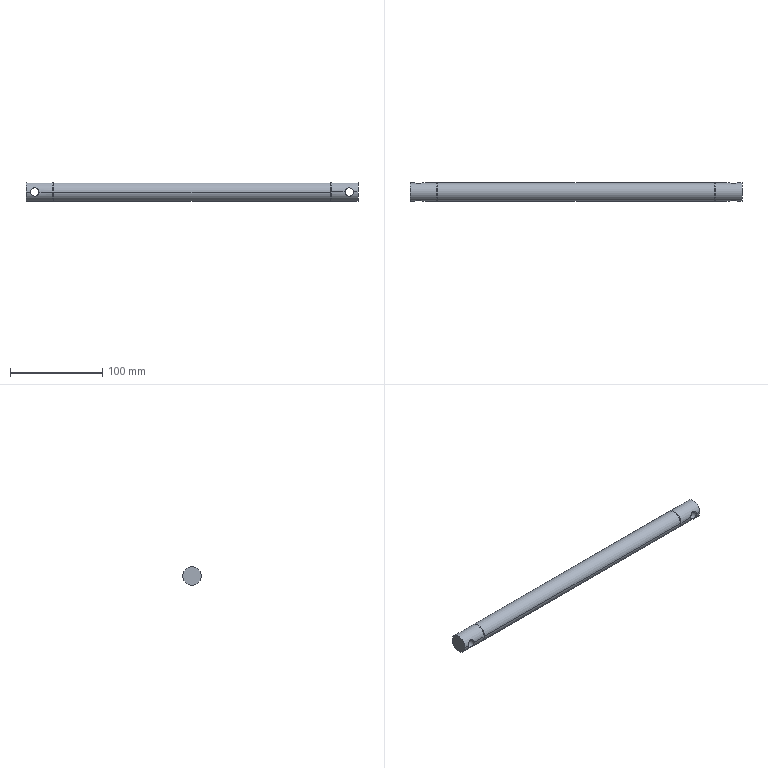Component | SolidWorks | DrivenShaft-1 | 1 solid | 20 faces | box 360 x 20 x 20 mm | volume 110558 mm3 | cylinder 14 | plane 6 | commonest cylinder face diameters 20 x6 9 x4 19 x4
build123d program:
from build123d import *

# Parameters (mm, degrees)
F_9_0_9_DIAMETER_HOLE1_D = 9


with BuildPart() as part:
    # Sketch1 → Revolve1 (revolve)
    with BuildSketch(Plane.XY, mode=Mode.PRIVATE) as revolve1_sk:
        Polygon((0, 0), (360, 0), (360, 10), (331, 10), (331, 9.5), (330, 9.5), (330, 10), (30, 10), (30, 9.5), (29, 9.5), (29, 10), (0, 10), align=None)
    revolve(revolve1_sk.sketch.rotate(Axis((0, 0, 0), (1, 0, 0)), 90), axis=Axis((0, 0, 0), (1, 0, 0)))

    # 9.0 _9_ Diameter Hole1 (through all)
    with Locations(Plane.XY.offset(10)):
        with Locations((9.5, 0), (350.5, 0)):
            Hole(F_9_0_9_DIAMETER_HOLE1_D / 2)


solid = part.part

# Placed as in the assembly
solid = solid.moved(Location((5755.006, 3057.679, 47.375), (90, 0, 0)))
STEP:
#1=COLOUR_RGB('',0.7922,0.8196,0.9333);
#2=FILL_AREA_STYLE_COLOUR('',#1);
#3=FILL_AREA_STYLE('',(#2));
#4=SURFACE_STYLE_FILL_AREA(#3);
#5=SURFACE_SIDE_STYLE('',(#4));
#6=SURFACE_STYLE_USAGE(.BOTH.,#5);
#7=PRESENTATION_STYLE_ASSIGNMENT((#6));
#8=CARTESIAN_POINT('',(240.551,119.987,1.865));
#9=VERTEX_POINT('',#8);
#10=CARTESIAN_POINT('',(240.197,119.987,1.865));
#11=VERTEX_POINT('',#10);
#12=CARTESIAN_POINT('',(240.551,119.987,1.865));
#13=CARTESIAN_POINT('',(240.551,119.987,1.853));
#14=CARTESIAN_POINT('',(240.55,119.988,1.842));
#15=CARTESIAN_POINT('',(240.546,119.99,1.819));
#16=CARTESIAN_POINT('',(240.542,119.991,1.808));
#17=CARTESIAN_POINT('',(240.533,119.995,1.786));
#18=CARTESIAN_POINT('',(240.528,119.998,1.776));
#19=CARTESIAN_POINT('',(240.515,120.002,1.757));
#20=CARTESIAN_POINT('',(240.508,120.005,1.748));
#21=CARTESIAN_POINT('',(240.491,120.011,1.732));
#22=CARTESIAN_POINT('',(240.482,120.013,1.724));
#23=CARTESIAN_POINT('',(240.463,120.018,1.712));
#24=CARTESIAN_POINT('',(240.453,120.021,1.706));
#25=CARTESIAN_POINT('',(240.432,120.025,1.697));
#26=CARTESIAN_POINT('',(240.421,120.027,1.694));
#27=CARTESIAN_POINT('',(240.404,120.028,1.69));
#28=CARTESIAN_POINT('',(240.398,120.029,1.689));
#29=CARTESIAN_POINT('',(240.386,120.029,1.688));
#30=CARTESIAN_POINT('',(240.38,120.029,1.688));
#31=CARTESIAN_POINT('',(240.363,120.029,1.688));
#32=CARTESIAN_POINT('',(240.351,120.029,1.689));
#33=CARTESIAN_POINT('',(240.328,120.027,1.694));
#34=CARTESIAN_POINT('',(240.317,120.025,1.697));
#35=CARTESIAN_POINT('',(240.295,120.021,1.706));
#36=CARTESIAN_POINT('',(240.285,120.018,1.712));
#37=CARTESIAN_POINT('',(240.266,120.013,1.724));
#38=CARTESIAN_POINT('',(240.257,120.011,1.732));
#39=CARTESIAN_POINT('',(240.241,120.005,1.748));
#40=CARTESIAN_POINT('',(240.234,120.002,1.757));
#41=CARTESIAN_POINT('',(240.221,119.998,1.776));
#42=CARTESIAN_POINT('',(240.215,119.995,1.786));
#43=CARTESIAN_POINT('',(240.206,119.991,1.807));
#44=CARTESIAN_POINT('',(240.203,119.99,1.819));
#45=CARTESIAN_POINT('',(240.198,119.988,1.841));
#46=CARTESIAN_POINT('',(240.197,119.987,1.853));
#47=CARTESIAN_POINT('',(240.197,119.987,1.865));
#48=B_SPLINE_CURVE_WITH_KNOTS('',3,(#12,#13,#14,#15,#16,#17,#18,#19,#20,#21,#22,#23,#24,#25,#26,#27,#28,#29,#30,#31,#32,#33,#34,#35,#36,#37,#38,#39,#40,#41,#42,#43,#44,#45,#46,#47),.UNSPECIFIED.,.F.,.F.,(4,2,2,2,2,2,2,2,2,2,2,2,2,2,2,2,2,4),(0.01426,0.01515,0.01604,0.01693,0.01783,0.01872,0.01961,0.0205,0.02094,0.02139,0.02228,0.02317,0.02406,0.02495,0.02584,0.02673,0.02762,0.02851),.UNSPECIFIED.);
#49=EDGE_CURVE('',#9,#11,#48,.T.);
#50=ORIENTED_EDGE('',*,*,#49,.F.);
#51=CARTESIAN_POINT('',(240.551,120.775,1.865));
#52=VERTEX_POINT('',#51);
#53=CARTESIAN_POINT('',(240.551,120.775,1.865));
#54=DIRECTION('',(-0.,1.,0.));
#55=VECTOR('',#54,39.37);
#56=LINE('',#53,#55);
#57=EDGE_CURVE('',#9,#52,#56,.T.);
#58=ORIENTED_EDGE('',*,*,#57,.T.);
#59=CARTESIAN_POINT('',(240.197,120.775,1.865));
#60=VERTEX_POINT('',#59);
#61=CARTESIAN_POINT('',(240.197,120.775,1.865));
#62=CARTESIAN_POINT('',(240.197,120.775,1.853));
#63=CARTESIAN_POINT('',(240.198,120.774,1.842));
#64=CARTESIAN_POINT('',(240.203,120.772,1.819));
#65=CARTESIAN_POINT('',(240.206,120.771,1.807));
#66=CARTESIAN_POINT('',(240.215,120.767,1.786));
#67=CARTESIAN_POINT('',(240.221,120.765,1.776));
#68=CARTESIAN_POINT('',(240.234,120.76,1.757));
#69=CARTESIAN_POINT('',(240.241,120.757,1.748));
#70=CARTESIAN_POINT('',(240.257,120.752,1.732));
#71=CARTESIAN_POINT('',(240.266,120.749,1.724));
#72=CARTESIAN_POINT('',(240.285,120.744,1.712));
#73=CARTESIAN_POINT('',(240.295,120.741,1.706));
#74=CARTESIAN_POINT('',(240.311,120.738,1.699));
#75=CARTESIAN_POINT('',(240.317,120.737,1.698));
#76=CARTESIAN_POINT('',(240.328,120.736,1.694));
#77=CARTESIAN_POINT('',(240.334,120.735,1.693));
#78=CARTESIAN_POINT('',(240.351,120.733,1.689));
#79=CARTESIAN_POINT('',(240.362,120.733,1.688));
#80=CARTESIAN_POINT('',(240.386,120.733,1.688));
#81=CARTESIAN_POINT('',(240.398,120.733,1.689));
#82=CARTESIAN_POINT('',(240.421,120.736,1.694));
#83=CARTESIAN_POINT('',(240.432,120.737,1.697));
#84=CARTESIAN_POINT('',(240.453,120.741,1.706));
#85=CARTESIAN_POINT('',(240.463,120.744,1.712));
#86=CARTESIAN_POINT('',(240.483,120.749,1.724));
#87=CARTESIAN_POINT('',(240.492,120.752,1.732));
#88=CARTESIAN_POINT('',(240.508,120.757,1.748));
#89=CARTESIAN_POINT('',(240.515,120.76,1.757));
#90=CARTESIAN_POINT('',(240.528,120.765,1.776));
#91=CARTESIAN_POINT('',(240.533,120.767,1.786));
#92=CARTESIAN_POINT('',(240.542,120.771,1.807));
#93=CARTESIAN_POINT('',(240.546,120.772,1.819));
#94=CARTESIAN_POINT('',(240.55,120.774,1.842));
#95=CARTESIAN_POINT('',(240.551,120.775,1.853));
#96=CARTESIAN_POINT('',(240.551,120.775,1.865));
#97=B_SPLINE_CURVE_WITH_KNOTS('',3,(#61,#62,#63,#64,#65,#66,#67,#68,#69,#70,#71,#72,#73,#74,#75,#76,#77,#78,#79,#80,#81,#82,#83,#84,#85,#86,#87,#88,#89,#90,#91,#92,#93,#94,#95,#96),.UNSPECIFIED.,.F.,.F.,(4,2,2,2,2,2,2,2,2,2,2,2,2,2,2,2,2,4),(0.,0.0008915,0.001783,0.002674,0.003566,0.004457,0.005349,0.005794,0.00624,0.007132,0.008023,0.008915,0.009806,0.0107,0.01159,0.01248,0.01337,0.01426),.UNSPECIFIED.);
#98=EDGE_CURVE('',#60,#52,#97,.T.);
#99=ORIENTED_EDGE('',*,*,#98,.F.);
#100=CARTESIAN_POINT('',(240.197,120.775,1.865));
#101=DIRECTION('',(-0.,1.,0.));
#102=VECTOR('',#101,39.37);
#103=LINE('',#100,#102);
#104=EDGE_CURVE('',#11,#60,#103,.T.);
#105=ORIENTED_EDGE('',*,*,#104,.F.);
#106=EDGE_LOOP('',(#50,#58,#99,#105));
#107=FACE_OUTER_BOUND('',#106,.T.);
#108=CARTESIAN_POINT('',(240.374,120.775,1.865));
#109=DIRECTION('',(-0.,1.,0.));
#110=DIRECTION('',(-1.,0.,0.));
#111=AXIS2_PLACEMENT_3D('',#108,#109,#110);
#112=CYLINDRICAL_SURFACE('',#111,0.1772);
#113=ADVANCED_FACE('',(#107),#112,.F.);
#114=CARTESIAN_POINT('',(227.126,119.987,1.865));
#115=VERTEX_POINT('',#114);
#116=CARTESIAN_POINT('',(226.772,119.987,1.865));
#117=VERTEX_POINT('',#116);
#118=CARTESIAN_POINT('',(227.126,119.987,1.865));
#119=CARTESIAN_POINT('',(227.126,119.987,1.853));
#120=CARTESIAN_POINT('',(227.125,119.988,1.842));
#121=CARTESIAN_POINT('',(227.12,119.99,1.819));
#122=CARTESIAN_POINT('',(227.117,119.991,1.808));
#123=CARTESIAN_POINT('',(227.108,119.995,1.786));
#124=CARTESIAN_POINT('',(227.102,119.998,1.776));
#125=CARTESIAN_POINT('',(227.09,120.002,1.757));
#126=CARTESIAN_POINT('',(227.082,120.005,1.748));
#127=CARTESIAN_POINT('',(227.066,120.011,1.732));
#128=CARTESIAN_POINT('',(227.057,120.013,1.724));
#129=CARTESIAN_POINT('',(227.038,120.018,1.712));
#130=CARTESIAN_POINT('',(227.028,120.021,1.706));
#131=CARTESIAN_POINT('',(227.007,120.025,1.697));
#132=CARTESIAN_POINT('',(226.996,120.027,1.694));
#133=CARTESIAN_POINT('',(226.978,120.028,1.69));
#134=CARTESIAN_POINT('',(226.973,120.029,1.689));
#135=CARTESIAN_POINT('',(226.961,120.029,1.688));
#136=CARTESIAN_POINT('',(226.955,120.029,1.688));
#137=CARTESIAN_POINT('',(226.937,120.029,1.688));
#138=CARTESIAN_POINT('',(226.926,120.029,1.689));
#139=CARTESIAN_POINT('',(226.903,120.027,1.694));
#140=CARTESIAN_POINT('',(226.892,120.025,1.697));
#141=CARTESIAN_POINT('',(226.87,120.021,1.706));
#142=CARTESIAN_POINT('',(226.86,120.018,1.712));
#143=CARTESIAN_POINT('',(226.841,120.013,1.724));
#144=CARTESIAN_POINT('',(226.832,120.011,1.732));
#145=CARTESIAN_POINT('',(226.816,120.005,1.748));
#146=CARTESIAN_POINT('',(226.808,120.002,1.757));
#147=CARTESIAN_POINT('',(226.796,119.998,1.776));
#148=CARTESIAN_POINT('',(226.79,119.995,1.786));
#149=CARTESIAN_POINT('',(226.781,119.991,1.807));
#150=CARTESIAN_POINT('',(226.778,119.99,1.819));
#151=CARTESIAN_POINT('',(226.773,119.988,1.841));
#152=CARTESIAN_POINT('',(226.772,119.987,1.853));
#153=CARTESIAN_POINT('',(226.772,119.987,1.865));
#154=B_SPLINE_CURVE_WITH_KNOTS('',3,(#118,#119,#120,#121,#122,#123,#124,#125,#126,#127,#128,#129,#130,#131,#132,#133,#134,#135,#136,#137,#138,#139,#140,#141,#142,#143,#144,#145,#146,#147,#148,#149,#150,#151,#152,#153),.UNSPECIFIED.,.F.,.F.,(4,2,2,2,2,2,2,2,2,2,2,2,2,2,2,2,2,4),(0.01426,0.01515,0.01604,0.01693,0.01783,0.01872,0.01961,0.0205,0.02094,0.02139,0.02228,0.02317,0.02406,0.02495,0.02584,0.02673,0.02762,0.02851),.UNSPECIFIED.);
#155=EDGE_CURVE('',#115,#117,#154,.T.);
#156=ORIENTED_EDGE('',*,*,#155,.F.);
#157=CARTESIAN_POINT('',(227.126,120.775,1.865));
#158=VERTEX_POINT('',#157);
#159=CARTESIAN_POINT('',(227.126,120.775,1.865));
#160=DIRECTION('',(-0.,1.,0.));
#161=VECTOR('',#160,39.37);
#162=LINE('',#159,#161);
#163=EDGE_CURVE('',#115,#158,#162,.T.);
#164=ORIENTED_EDGE('',*,*,#163,.T.);
#165=CARTESIAN_POINT('',(226.772,120.775,1.865));
#166=VERTEX_POINT('',#165);
#167=CARTESIAN_POINT('',(226.772,120.775,1.865));
#168=CARTESIAN_POINT('',(226.772,120.775,1.853));
#169=CARTESIAN_POINT('',(226.773,120.774,1.842));
#170=CARTESIAN_POINT('',(226.778,120.772,1.819));
#171=CARTESIAN_POINT('',(226.781,120.771,1.807));
#172=CARTESIAN_POINT('',(226.79,120.767,1.786));
#173=CARTESIAN_POINT('',(226.796,120.765,1.776));
#174=CARTESIAN_POINT('',(226.808,120.76,1.757));
#175=CARTESIAN_POINT('',(226.816,120.757,1.748));
#176=CARTESIAN_POINT('',(226.832,120.752,1.732));
#177=CARTESIAN_POINT('',(226.841,120.749,1.724));
#178=CARTESIAN_POINT('',(226.86,120.744,1.712));
#179=CARTESIAN_POINT('',(226.87,120.741,1.706));
#180=CARTESIAN_POINT('',(226.886,120.738,1.699));
#181=CARTESIAN_POINT('',(226.891,120.737,1.698));
#182=CARTESIAN_POINT('',(226.903,120.736,1.694));
#183=CARTESIAN_POINT('',(226.908,120.735,1.693));
#184=CARTESIAN_POINT('',(226.926,120.733,1.689));
#185=CARTESIAN_POINT('',(226.937,120.733,1.688));
#186=CARTESIAN_POINT('',(226.961,120.733,1.688));
#187=CARTESIAN_POINT('',(226.973,120.733,1.689));
#188=CARTESIAN_POINT('',(226.995,120.736,1.694));
#189=CARTESIAN_POINT('',(227.007,120.737,1.697));
#190=CARTESIAN_POINT('',(227.028,120.741,1.706));
#191=CARTESIAN_POINT('',(227.038,120.744,1.712));
#192=CARTESIAN_POINT('',(227.057,120.749,1.724));
#193=CARTESIAN_POINT('',(227.066,120.752,1.732));
#194=CARTESIAN_POINT('',(227.082,120.757,1.748));
#195=CARTESIAN_POINT('',(227.09,120.76,1.757));
#196=CARTESIAN_POINT('',(227.103,120.765,1.776));
#197=CARTESIAN_POINT('',(227.108,120.767,1.786));
#198=CARTESIAN_POINT('',(227.117,120.771,1.807));
#199=CARTESIAN_POINT('',(227.12,120.772,1.819));
#200=CARTESIAN_POINT('',(227.125,120.774,1.842));
#201=CARTESIAN_POINT('',(227.126,120.775,1.853));
#202=CARTESIAN_POINT('',(227.126,120.775,1.865));
#203=B_SPLINE_CURVE_WITH_KNOTS('',3,(#167,#168,#169,#170,#171,#172,#173,#174,#175,#176,#177,#178,#179,#180,#181,#182,#183,#184,#185,#186,#187,#188,#189,#190,#191,#192,#193,#194,#195,#196,#197,#198,#199,#200,#201,#202),.UNSPECIFIED.,.F.,.F.,(4,2,2,2,2,2,2,2,2,2,2,2,2,2,2,2,2,4),(0.,0.0008915,0.001783,0.002674,0.003566,0.004457,0.005349,0.005794,0.00624,0.007132,0.008023,0.008915,0.009806,0.0107,0.01159,0.01248,0.01337,0.01426),.UNSPECIFIED.);
#204=EDGE_CURVE('',#166,#158,#203,.T.);
#205=ORIENTED_EDGE('',*,*,#204,.F.);
#206=CARTESIAN_POINT('',(226.772,120.775,1.865));
#207=DIRECTION('',(-0.,1.,0.));
#208=VECTOR('',#207,39.37);
#209=LINE('',#206,#208);
#210=EDGE_CURVE('',#117,#166,#209,.T.);
#211=ORIENTED_EDGE('',*,*,#210,.F.);
#212=EDGE_LOOP('',(#156,#164,#205,#211));
#213=FACE_OUTER_BOUND('',#212,.T.);
#214=CARTESIAN_POINT('',(226.949,120.775,1.865));
#215=DIRECTION('',(-0.,1.,0.));
#216=DIRECTION('',(-1.,0.,0.));
#217=AXIS2_PLACEMENT_3D('',#214,#215,#216);
#218=CYLINDRICAL_SURFACE('',#217,0.1772);
#219=ADVANCED_FACE('',(#213),#218,.F.);
#220=CARTESIAN_POINT('',(226.575,120.775,1.865));
#221=VERTEX_POINT('',#220);
#222=CARTESIAN_POINT('',(226.575,119.987,1.865));
#223=VERTEX_POINT('',#222);
#224=CARTESIAN_POINT('',(226.575,120.381,1.865));
#225=DIRECTION('',(1.,0.,0.));
#226=DIRECTION('',(0.,1.,0.));
#227=AXIS2_PLACEMENT_3D('',#224,#225,#226);
#228=CIRCLE('',#227,0.3937);
#229=EDGE_CURVE('',#221,#223,#228,.T.);
#230=ORIENTED_EDGE('',*,*,#229,.T.);
#231=CARTESIAN_POINT('',(240.748,119.987,1.865));
#232=DIRECTION('',(1.,0.,0.));
#233=VECTOR('',#232,39.37);
#234=LINE('',#231,#233);
#235=EDGE_CURVE('',#223,#117,#234,.T.);
#236=ORIENTED_EDGE('',*,*,#235,.T.);
#237=CARTESIAN_POINT('',(226.772,119.987,1.865));
#238=CARTESIAN_POINT('',(226.772,119.987,1.877));
#239=CARTESIAN_POINT('',(226.773,119.988,1.889));
#240=CARTESIAN_POINT('',(226.778,119.99,1.912));
#241=CARTESIAN_POINT('',(226.781,119.991,1.923));
#242=CARTESIAN_POINT('',(226.79,119.995,1.944));
#243=CARTESIAN_POINT('',(226.796,119.997,1.954));
#244=CARTESIAN_POINT('',(226.808,120.002,1.974));
#245=CARTESIAN_POINT('',(226.816,120.005,1.982));
#246=CARTESIAN_POINT('',(226.832,120.011,1.999));
#247=CARTESIAN_POINT('',(226.841,120.013,2.006));
#248=CARTESIAN_POINT('',(226.86,120.019,2.019));
#249=CARTESIAN_POINT('',(226.87,120.021,2.024));
#250=CARTESIAN_POINT('',(226.886,120.024,2.031));
#251=CARTESIAN_POINT('',(226.891,120.025,2.033));
#252=CARTESIAN_POINT('',(226.903,120.026,2.036));
#253=CARTESIAN_POINT('',(226.908,120.027,2.038));
#254=CARTESIAN_POINT('',(226.926,120.029,2.041));
#255=CARTESIAN_POINT('',(226.937,120.029,2.042));
#256=CARTESIAN_POINT('',(226.961,120.029,2.042));
#257=CARTESIAN_POINT('',(226.973,120.029,2.041));
#258=CARTESIAN_POINT('',(226.995,120.027,2.037));
#259=CARTESIAN_POINT('',(227.007,120.025,2.033));
#260=CARTESIAN_POINT('',(227.028,120.021,2.024));
#261=CARTESIAN_POINT('',(227.038,120.018,2.019));
#262=CARTESIAN_POINT('',(227.057,120.013,2.006));
#263=CARTESIAN_POINT('',(227.066,120.011,1.998));
#264=CARTESIAN_POINT('',(227.082,120.005,1.982));
#265=CARTESIAN_POINT('',(227.09,120.002,1.974));
#266=CARTESIAN_POINT('',(227.103,119.997,1.954));
#267=CARTESIAN_POINT('',(227.108,119.995,1.944));
#268=CARTESIAN_POINT('',(227.117,119.991,1.923));
#269=CARTESIAN_POINT('',(227.12,119.99,1.912));
#270=CARTESIAN_POINT('',(227.125,119.988,1.889));
#271=CARTESIAN_POINT('',(227.126,119.987,1.877));
#272=CARTESIAN_POINT('',(227.126,119.987,1.865));
#273=B_SPLINE_CURVE_WITH_KNOTS('',3,(#237,#238,#239,#240,#241,#242,#243,#244,#245,#246,#247,#248,#249,#250,#251,#252,#253,#254,#255,#256,#257,#258,#259,#260,#261,#262,#263,#264,#265,#266,#267,#268,#269,#270,#271,#272),.UNSPECIFIED.,.F.,.F.,(4,2,2,2,2,2,2,2,2,2,2,2,2,2,2,2,2,4),(0.,0.0008915,0.001783,0.002674,0.003566,0.004457,0.005349,0.005794,0.00624,0.007132,0.008023,0.008915,0.009806,0.0107,0.01159,0.01248,0.01337,0.01426),.UNSPECIFIED.);
#274=EDGE_CURVE('',#117,#115,#273,.T.);
#275=ORIENTED_EDGE('',*,*,#274,.T.);
#276=CARTESIAN_POINT('',(227.717,119.987,1.865));
#277=VERTEX_POINT('',#276);
#278=CARTESIAN_POINT('',(240.748,119.987,1.865));
#279=DIRECTION('',(1.,0.,0.));
#280=VECTOR('',#279,39.37);
#281=LINE('',#278,#280);
#282=EDGE_CURVE('',#115,#277,#281,.T.);
#283=ORIENTED_EDGE('',*,*,#282,.T.);
#284=CARTESIAN_POINT('',(227.717,120.775,1.865));
#285=VERTEX_POINT('',#284);
#286=CARTESIAN_POINT('',(227.717,120.381,1.865));
#287=DIRECTION('',(1.,0.,0.));
#288=DIRECTION('',(0.,1.,0.));
#289=AXIS2_PLACEMENT_3D('',#286,#287,#288);
#290=CIRCLE('',#289,0.3937);
#291=EDGE_CURVE('',#285,#277,#290,.T.);
#292=ORIENTED_EDGE('',*,*,#291,.F.);
#293=CARTESIAN_POINT('',(240.748,120.775,1.865));
#294=DIRECTION('',(1.,0.,0.));
#295=VECTOR('',#294,39.37);
#296=LINE('',#293,#295);
#297=EDGE_CURVE('',#158,#285,#296,.T.);
#298=ORIENTED_EDGE('',*,*,#297,.F.);
#299=CARTESIAN_POINT('',(227.126,120.775,1.865));
#300=CARTESIAN_POINT('',(227.126,120.775,1.877));
#301=CARTESIAN_POINT('',(227.125,120.774,1.889));
#302=CARTESIAN_POINT('',(227.12,120.772,1.912));
#303=CARTESIAN_POINT('',(227.117,120.771,1.923));
#304=CARTESIAN_POINT('',(227.108,120.767,1.944));
#305=CARTESIAN_POINT('',(227.102,120.765,1.955));
#306=CARTESIAN_POINT('',(227.09,120.76,1.974));
#307=CARTESIAN_POINT('',(227.082,120.757,1.982));
#308=CARTESIAN_POINT('',(227.066,120.752,1.999));
#309=CARTESIAN_POINT('',(227.057,120.749,2.006));
#310=CARTESIAN_POINT('',(227.038,120.744,2.019));
#311=CARTESIAN_POINT('',(227.028,120.741,2.024));
#312=CARTESIAN_POINT('',(227.007,120.737,2.033));
#313=CARTESIAN_POINT('',(226.996,120.736,2.036));
#314=CARTESIAN_POINT('',(226.978,120.734,2.04));
#315=CARTESIAN_POINT('',(226.973,120.733,2.041));
#316=CARTESIAN_POINT('',(226.961,120.733,2.042));
#317=CARTESIAN_POINT('',(226.955,120.733,2.042));
#318=CARTESIAN_POINT('',(226.937,120.733,2.042));
#319=CARTESIAN_POINT('',(226.926,120.733,2.041));
#320=CARTESIAN_POINT('',(226.903,120.736,2.037));
#321=CARTESIAN_POINT('',(226.892,120.737,2.033));
#322=CARTESIAN_POINT('',(226.87,120.741,2.024));
#323=CARTESIAN_POINT('',(226.86,120.744,2.019));
#324=CARTESIAN_POINT('',(226.841,120.749,2.006));
#325=CARTESIAN_POINT('',(226.832,120.752,1.999));
#326=CARTESIAN_POINT('',(226.816,120.757,1.982));
#327=CARTESIAN_POINT('',(226.808,120.76,1.974));
#328=CARTESIAN_POINT('',(226.796,120.765,1.955));
#329=CARTESIAN_POINT('',(226.79,120.767,1.944));
#330=CARTESIAN_POINT('',(226.781,120.771,1.923));
#331=CARTESIAN_POINT('',(226.778,120.772,1.912));
#332=CARTESIAN_POINT('',(226.773,120.774,1.889));
#333=CARTESIAN_POINT('',(226.772,120.775,1.877));
#334=CARTESIAN_POINT('',(226.772,120.775,1.865));
#335=B_SPLINE_CURVE_WITH_KNOTS('',3,(#299,#300,#301,#302,#303,#304,#305,#306,#307,#308,#309,#310,#311,#312,#313,#314,#315,#316,#317,#318,#319,#320,#321,#322,#323,#324,#325,#326,#327,#328,#329,#330,#331,#332,#333,#334),.UNSPECIFIED.,.F.,.F.,(4,2,2,2,2,2,2,2,2,2,2,2,2,2,2,2,2,4),(0.01426,0.01515,0.01604,0.01693,0.01783,0.01872,0.01961,0.0205,0.02094,0.02139,0.02228,0.02317,0.02406,0.02495,0.02584,0.02673,0.02762,0.02851),.UNSPECIFIED.);
#336=EDGE_CURVE('',#158,#166,#335,.T.);
#337=ORIENTED_EDGE('',*,*,#336,.T.);
#338=CARTESIAN_POINT('',(240.748,120.775,1.865));
#339=DIRECTION('',(1.,0.,0.));
#340=VECTOR('',#339,39.37);
#341=LINE('',#338,#340);
#342=EDGE_CURVE('',#221,#166,#341,.T.);
#343=ORIENTED_EDGE('',*,*,#342,.F.);
#344=EDGE_LOOP('',(#230,#236,#275,#283,#292,#298,#337,#343));
#345=FACE_OUTER_BOUND('',#344,.T.);
#346=CARTESIAN_POINT('',(240.748,120.381,1.865));
#347=DIRECTION('',(1.,0.,0.));
#348=DIRECTION('',(0.,1.,0.));
#349=AXIS2_PLACEMENT_3D('',#346,#347,#348);
#350=CYLINDRICAL_SURFACE('',#349,0.3937);
#351=ADVANCED_FACE('',(#345),#350,.T.);
#352=CARTESIAN_POINT('',(227.717,120.755,1.865));
#353=VERTEX_POINT('',#352);
#354=CARTESIAN_POINT('',(227.717,120.007,1.865));
#355=VERTEX_POINT('',#354);
#356=CARTESIAN_POINT('',(227.717,120.381,1.865));
#357=DIRECTION('',(1.,0.,0.));
#358=DIRECTION('',(0.,1.,0.));
#359=AXIS2_PLACEMENT_3D('',#356,#357,#358);
#360=CIRCLE('',#359,0.374);
#361=EDGE_CURVE('',#353,#355,#360,.T.);
#362=ORIENTED_EDGE('',*,*,#361,.T.);
#363=CARTESIAN_POINT('',(227.756,120.007,1.865));
#364=VERTEX_POINT('',#363);
#365=CARTESIAN_POINT('',(240.748,120.007,1.865));
#366=DIRECTION('',(1.,0.,0.));
#367=VECTOR('',#366,39.37);
#368=LINE('',#365,#367);
#369=EDGE_CURVE('',#355,#364,#368,.T.);
#370=ORIENTED_EDGE('',*,*,#369,.T.);
#371=CARTESIAN_POINT('',(227.756,120.755,1.865));
#372=VERTEX_POINT('',#371);
#373=CARTESIAN_POINT('',(227.756,120.381,1.865));
#374=DIRECTION('',(1.,0.,0.));
#375=DIRECTION('',(0.,1.,0.));
#376=AXIS2_PLACEMENT_3D('',#373,#374,#375);
#377=CIRCLE('',#376,0.374);
#378=EDGE_CURVE('',#372,#364,#377,.T.);
#379=ORIENTED_EDGE('',*,*,#378,.F.);
#380=CARTESIAN_POINT('',(240.748,120.755,1.865));
#381=DIRECTION('',(1.,0.,0.));
#382=VECTOR('',#381,39.37);
#383=LINE('',#380,#382);
#384=EDGE_CURVE('',#353,#372,#383,.T.);
#385=ORIENTED_EDGE('',*,*,#384,.F.);
#386=EDGE_LOOP('',(#362,#370,#379,#385));
#387=FACE_OUTER_BOUND('',#386,.T.);
#388=CARTESIAN_POINT('',(240.748,120.381,1.865));
#389=DIRECTION('',(1.,0.,0.));
#390=DIRECTION('',(0.,1.,0.));
#391=AXIS2_PLACEMENT_3D('',#388,#389,#390);
#392=CYLINDRICAL_SURFACE('',#391,0.374);
#393=ADVANCED_FACE('',(#387),#392,.T.);
#394=CARTESIAN_POINT('',(227.756,120.775,1.865));
#395=VERTEX_POINT('',#394);
#396=CARTESIAN_POINT('',(227.756,119.987,1.865));
#397=VERTEX_POINT('',#396);
#398=CARTESIAN_POINT('',(227.756,120.381,1.865));
#399=DIRECTION('',(1.,0.,0.));
#400=DIRECTION('',(0.,1.,0.));
#401=AXIS2_PLACEMENT_3D('',#398,#399,#400);
#402=CIRCLE('',#401,0.3937);
#403=EDGE_CURVE('',#395,#397,#402,.T.);
#404=ORIENTED_EDGE('',*,*,#403,.T.);
#405=CARTESIAN_POINT('',(239.567,119.987,1.865));
#406=VERTEX_POINT('',#405);
#407=CARTESIAN_POINT('',(240.748,119.987,1.865));
#408=DIRECTION('',(1.,0.,0.));
#409=VECTOR('',#408,39.37);
#410=LINE('',#407,#409);
#411=EDGE_CURVE('',#397,#406,#410,.T.);
#412=ORIENTED_EDGE('',*,*,#411,.T.);
#413=CARTESIAN_POINT('',(239.567,120.775,1.865));
#414=VERTEX_POINT('',#413);
#415=CARTESIAN_POINT('',(239.567,120.381,1.865));
#416=DIRECTION('',(1.,0.,0.));
#417=DIRECTION('',(0.,1.,0.));
#418=AXIS2_PLACEMENT_3D('',#415,#416,#417);
#419=CIRCLE('',#418,0.3937);
#420=EDGE_CURVE('',#414,#406,#419,.T.);
#421=ORIENTED_EDGE('',*,*,#420,.F.);
#422=CARTESIAN_POINT('',(240.748,120.775,1.865));
#423=DIRECTION('',(1.,0.,0.));
#424=VECTOR('',#423,39.37);
#425=LINE('',#422,#424);
#426=EDGE_CURVE('',#395,#414,#425,.T.);
#427=ORIENTED_EDGE('',*,*,#426,.F.);
#428=EDGE_LOOP('',(#404,#412,#421,#427));
#429=FACE_OUTER_BOUND('',#428,.T.);
#430=CARTESIAN_POINT('',(240.748,120.381,1.865));
#431=DIRECTION('',(1.,0.,0.));
#432=DIRECTION('',(0.,1.,0.));
#433=AXIS2_PLACEMENT_3D('',#430,#431,#432);
#434=CYLINDRICAL_SURFACE('',#433,0.3937);
#435=ADVANCED_FACE('',(#429),#434,.T.);
#436=CARTESIAN_POINT('',(239.567,120.755,1.865));
#437=VERTEX_POINT('',#436);
#438=CARTESIAN_POINT('',(239.567,120.007,1.865));
#439=VERTEX_POINT('',#438);
#440=CARTESIAN_POINT('',(239.567,120.381,1.865));
#441=DIRECTION('',(1.,0.,0.));
#442=DIRECTION('',(0.,1.,0.));
#443=AXIS2_PLACEMENT_3D('',#440,#441,#442);
#444=CIRCLE('',#443,0.374);
#445=EDGE_CURVE('',#437,#439,#444,.T.);
#446=ORIENTED_EDGE('',*,*,#445,.T.);
#447=CARTESIAN_POINT('',(239.607,120.007,1.865));
#448=VERTEX_POINT('',#447);
#449=CARTESIAN_POINT('',(240.748,120.007,1.865));
#450=DIRECTION('',(1.,0.,0.));
#451=VECTOR('',#450,39.37);
#452=LINE('',#449,#451);
#453=EDGE_CURVE('',#439,#448,#452,.T.);
#454=ORIENTED_EDGE('',*,*,#453,.T.);
#455=CARTESIAN_POINT('',(239.607,120.755,1.865));
#456=VERTEX_POINT('',#455);
#457=CARTESIAN_POINT('',(239.607,120.381,1.865));
#458=DIRECTION('',(1.,0.,0.));
#459=DIRECTION('',(0.,1.,0.));
#460=AXIS2_PLACEMENT_3D('',#457,#458,#459);
#461=CIRCLE('',#460,0.374);
#462=EDGE_CURVE('',#456,#448,#461,.T.);
#463=ORIENTED_EDGE('',*,*,#462,.F.);
#464=CARTESIAN_POINT('',(240.748,120.755,1.865));
#465=DIRECTION('',(1.,0.,0.));
#466=VECTOR('',#465,39.37);
#467=LINE('',#464,#466);
#468=EDGE_CURVE('',#437,#456,#467,.T.);
#469=ORIENTED_EDGE('',*,*,#468,.F.);
#470=EDGE_LOOP('',(#446,#454,#463,#469));
#471=FACE_OUTER_BOUND('',#470,.T.);
#472=CARTESIAN_POINT('',(240.748,120.381,1.865));
#473=DIRECTION('',(1.,0.,0.));
#474=DIRECTION('',(0.,1.,0.));
#475=AXIS2_PLACEMENT_3D('',#472,#473,#474);
#476=CYLINDRICAL_SURFACE('',#475,0.374);
#477=ADVANCED_FACE('',(#471),#476,.T.);
#478=CARTESIAN_POINT('',(239.607,120.775,1.865));
#479=VERTEX_POINT('',#478);
#480=CARTESIAN_POINT('',(239.607,119.987,1.865));
#481=VERTEX_POINT('',#480);
#482=CARTESIAN_POINT('',(239.607,120.381,1.865));
#483=DIRECTION('',(1.,0.,0.));
#484=DIRECTION('',(0.,1.,0.));
#485=AXIS2_PLACEMENT_3D('',#482,#483,#484);
#486=CIRCLE('',#485,0.3937);
#487=EDGE_CURVE('',#479,#481,#486,.T.);
#488=ORIENTED_EDGE('',*,*,#487,.T.);
#489=CARTESIAN_POINT('',(240.748,119.987,1.865));
#490=DIRECTION('',(1.,0.,0.));
#491=VECTOR('',#490,39.37);
#492=LINE('',#489,#491);
#493=EDGE_CURVE('',#481,#11,#492,.T.);
#494=ORIENTED_EDGE('',*,*,#493,.T.);
#495=CARTESIAN_POINT('',(240.197,119.987,1.865));
#496=CARTESIAN_POINT('',(240.197,119.987,1.877));
#497=CARTESIAN_POINT('',(240.198,119.988,1.889));
#498=CARTESIAN_POINT('',(240.203,119.99,1.912));
#499=CARTESIAN_POINT('',(240.206,119.991,1.923));
#500=CARTESIAN_POINT('',(240.215,119.995,1.944));
#501=CARTESIAN_POINT('',(240.221,119.997,1.954));
#502=CARTESIAN_POINT('',(240.234,120.002,1.974));
#503=CARTESIAN_POINT('',(240.241,120.005,1.982));
#504=CARTESIAN_POINT('',(240.257,120.011,1.999));
#505=CARTESIAN_POINT('',(240.266,120.013,2.006));
#506=CARTESIAN_POINT('',(240.285,120.019,2.019));
#507=CARTESIAN_POINT('',(240.295,120.021,2.024));
#508=CARTESIAN_POINT('',(240.311,120.024,2.031));
#509=CARTESIAN_POINT('',(240.317,120.025,2.033));
#510=CARTESIAN_POINT('',(240.328,120.026,2.036));
#511=CARTESIAN_POINT('',(240.334,120.027,2.038));
#512=CARTESIAN_POINT('',(240.351,120.029,2.041));
#513=CARTESIAN_POINT('',(240.362,120.029,2.042));
#514=CARTESIAN_POINT('',(240.386,120.029,2.042));
#515=CARTESIAN_POINT('',(240.398,120.029,2.041));
#516=CARTESIAN_POINT('',(240.421,120.027,2.037));
#517=CARTESIAN_POINT('',(240.432,120.025,2.033));
#518=CARTESIAN_POINT('',(240.453,120.021,2.024));
#519=CARTESIAN_POINT('',(240.463,120.018,2.019));
#520=CARTESIAN_POINT('',(240.483,120.013,2.006));
#521=CARTESIAN_POINT('',(240.492,120.011,1.998));
#522=CARTESIAN_POINT('',(240.508,120.005,1.982));
#523=CARTESIAN_POINT('',(240.515,120.002,1.974));
#524=CARTESIAN_POINT('',(240.528,119.997,1.954));
#525=CARTESIAN_POINT('',(240.533,119.995,1.944));
#526=CARTESIAN_POINT('',(240.542,119.991,1.923));
#527=CARTESIAN_POINT('',(240.546,119.99,1.912));
#528=CARTESIAN_POINT('',(240.55,119.988,1.889));
#529=CARTESIAN_POINT('',(240.551,119.987,1.877));
#530=CARTESIAN_POINT('',(240.551,119.987,1.865));
#531=B_SPLINE_CURVE_WITH_KNOTS('',3,(#495,#496,#497,#498,#499,#500,#501,#502,#503,#504,#505,#506,#507,#508,#509,#510,#511,#512,#513,#514,#515,#516,#517,#518,#519,#520,#521,#522,#523,#524,#525,#526,#527,#528,#529,#530),.UNSPECIFIED.,.F.,.F.,(4,2,2,2,2,2,2,2,2,2,2,2,2,2,2,2,2,4),(0.,0.0008915,0.001783,0.002674,0.003566,0.004457,0.005349,0.005794,0.00624,0.007132,0.008023,0.008915,0.009806,0.0107,0.01159,0.01248,0.01337,0.01426),.UNSPECIFIED.);
#532=EDGE_CURVE('',#11,#9,#531,.T.);
#533=ORIENTED_EDGE('',*,*,#532,.T.);
#534=CARTESIAN_POINT('',(240.748,119.987,1.865));
#535=VERTEX_POINT('',#534);
#536=CARTESIAN_POINT('',(240.748,119.987,1.865));
#537=DIRECTION('',(1.,0.,0.));
#538=VECTOR('',#537,39.37);
#539=LINE('',#536,#538);
#540=EDGE_CURVE('',#9,#535,#539,.T.);
#541=ORIENTED_EDGE('',*,*,#540,.T.);
#542=CARTESIAN_POINT('',(240.748,120.775,1.865));
#543=VERTEX_POINT('',#542);
#544=CARTESIAN_POINT('',(240.748,120.381,1.865));
#545=DIRECTION('',(1.,0.,0.));
#546=DIRECTION('',(0.,1.,0.));
#547=AXIS2_PLACEMENT_3D('',#544,#545,#546);
#548=CIRCLE('',#547,0.3937);
#549=EDGE_CURVE('',#543,#535,#548,.T.);
#550=ORIENTED_EDGE('',*,*,#549,.F.);
#551=CARTESIAN_POINT('',(240.748,120.775,1.865));
#552=DIRECTION('',(1.,0.,0.));
#553=VECTOR('',#552,39.37);
#554=LINE('',#551,#553);
#555=EDGE_CURVE('',#52,#543,#554,.T.);
#556=ORIENTED_EDGE('',*,*,#555,.F.);
#557=CARTESIAN_POINT('',(240.551,120.775,1.865));
#558=CARTESIAN_POINT('',(240.551,120.775,1.877));
#559=CARTESIAN_POINT('',(240.55,120.774,1.889));
#560=CARTESIAN_POINT('',(240.546,120.772,1.912));
#561=CARTESIAN_POINT('',(240.542,120.771,1.923));
#562=CARTESIAN_POINT('',(240.533,120.767,1.944));
#563=CARTESIAN_POINT('',(240.528,120.765,1.955));
#564=CARTESIAN_POINT('',(240.515,120.76,1.974));
#565=CARTESIAN_POINT('',(240.508,120.757,1.982));
#566=CARTESIAN_POINT('',(240.491,120.752,1.999));
#567=CARTESIAN_POINT('',(240.482,120.749,2.006));
#568=CARTESIAN_POINT('',(240.463,120.744,2.019));
#569=CARTESIAN_POINT('',(240.453,120.741,2.024));
#570=CARTESIAN_POINT('',(240.432,120.737,2.033));
#571=CARTESIAN_POINT('',(240.421,120.736,2.036));
#572=CARTESIAN_POINT('',(240.404,120.734,2.04));
#573=CARTESIAN_POINT('',(240.398,120.733,2.041));
#574=CARTESIAN_POINT('',(240.386,120.733,2.042));
#575=CARTESIAN_POINT('',(240.38,120.733,2.042));
#576=CARTESIAN_POINT('',(240.363,120.733,2.042));
#577=CARTESIAN_POINT('',(240.351,120.733,2.041));
#578=CARTESIAN_POINT('',(240.328,120.736,2.037));
#579=CARTESIAN_POINT('',(240.317,120.737,2.033));
#580=CARTESIAN_POINT('',(240.295,120.741,2.024));
#581=CARTESIAN_POINT('',(240.285,120.744,2.019));
#582=CARTESIAN_POINT('',(240.266,120.749,2.006));
#583=CARTESIAN_POINT('',(240.257,120.752,1.999));
#584=CARTESIAN_POINT('',(240.241,120.757,1.982));
#585=CARTESIAN_POINT('',(240.234,120.76,1.974));
#586=CARTESIAN_POINT('',(240.221,120.765,1.955));
#587=CARTESIAN_POINT('',(240.215,120.767,1.944));
#588=CARTESIAN_POINT('',(240.206,120.771,1.923));
#589=CARTESIAN_POINT('',(240.203,120.772,1.912));
#590=CARTESIAN_POINT('',(240.198,120.774,1.889));
#591=CARTESIAN_POINT('',(240.197,120.775,1.877));
#592=CARTESIAN_POINT('',(240.197,120.775,1.865));
#593=B_SPLINE_CURVE_WITH_KNOTS('',3,(#557,#558,#559,#560,#561,#562,#563,#564,#565,#566,#567,#568,#569,#570,#571,#572,#573,#574,#575,#576,#577,#578,#579,#580,#581,#582,#583,#584,#585,#586,#587,#588,#589,#590,#591,#592),.UNSPECIFIED.,.F.,.F.,(4,2,2,2,2,2,2,2,2,2,2,2,2,2,2,2,2,4),(0.01426,0.01515,0.01604,0.01693,0.01783,0.01872,0.01961,0.0205,0.02094,0.02139,0.02228,0.02317,0.02406,0.02495,0.02584,0.02673,0.02762,0.02851),.UNSPECIFIED.);
#594=EDGE_CURVE('',#52,#60,#593,.T.);
#595=ORIENTED_EDGE('',*,*,#594,.T.);
#596=CARTESIAN_POINT('',(240.748,120.775,1.865));
#597=DIRECTION('',(1.,0.,0.));
#598=VECTOR('',#597,39.37);
#599=LINE('',#596,#598);
#600=EDGE_CURVE('',#479,#60,#599,.T.);
#601=ORIENTED_EDGE('',*,*,#600,.F.);
#602=EDGE_LOOP('',(#488,#494,#533,#541,#550,#556,#595,#601));
#603=FACE_OUTER_BOUND('',#602,.T.);
#604=CARTESIAN_POINT('',(240.748,120.381,1.865));
#605=DIRECTION('',(1.,0.,0.));
#606=DIRECTION('',(0.,1.,0.));
#607=AXIS2_PLACEMENT_3D('',#604,#605,#606);
#608=CYLINDRICAL_SURFACE('',#607,0.3937);
#609=ADVANCED_FACE('',(#603),#608,.T.);
#610=ORIENTED_EDGE('',*,*,#549,.T.);
#611=CARTESIAN_POINT('',(240.748,120.381,1.865));
#612=DIRECTION('',(1.,0.,0.));
#613=DIRECTION('',(0.,1.,0.));
#614=AXIS2_PLACEMENT_3D('',#611,#612,#613);
#615=CIRCLE('',#614,0.3937);
#616=EDGE_CURVE('',#535,#543,#615,.T.);
#617=ORIENTED_EDGE('',*,*,#616,.T.);
#618=EDGE_LOOP('',(#610,#617));
#619=FACE_OUTER_BOUND('',#618,.T.);
#620=CARTESIAN_POINT('',(240.748,120.381,1.865));
#621=DIRECTION('',(-1.,-0.,-0.));
#622=DIRECTION('',(0.,-1.,-0.));
#623=AXIS2_PLACEMENT_3D('',#620,#621,#622);
#624=PLANE('',#623);
#625=ADVANCED_FACE('',(#619),#624,.F.);
#626=ORIENTED_EDGE('',*,*,#493,.F.);
#627=CARTESIAN_POINT('',(239.607,120.381,1.865));
#628=DIRECTION('',(1.,0.,0.));
#629=DIRECTION('',(0.,1.,0.));
#630=AXIS2_PLACEMENT_3D('',#627,#628,#629);
#631=CIRCLE('',#630,0.3937);
#632=EDGE_CURVE('',#481,#479,#631,.T.);
#633=ORIENTED_EDGE('',*,*,#632,.T.);
#634=ORIENTED_EDGE('',*,*,#600,.T.);
#635=ORIENTED_EDGE('',*,*,#98,.T.);
#636=ORIENTED_EDGE('',*,*,#555,.T.);
#637=ORIENTED_EDGE('',*,*,#616,.F.);
#638=ORIENTED_EDGE('',*,*,#540,.F.);
#639=ORIENTED_EDGE('',*,*,#49,.T.);
#640=EDGE_LOOP('',(#626,#633,#634,#635,#636,#637,#638,#639));
#641=FACE_OUTER_BOUND('',#640,.T.);
#642=CARTESIAN_POINT('',(240.748,120.381,1.865));
#643=DIRECTION('',(1.,0.,0.));
#644=DIRECTION('',(0.,1.,0.));
#645=AXIS2_PLACEMENT_3D('',#642,#643,#644);
#646=CYLINDRICAL_SURFACE('',#645,0.3937);
#647=ADVANCED_FACE('',(#641),#646,.T.);
#648=ORIENTED_EDGE('',*,*,#487,.F.);
#649=ORIENTED_EDGE('',*,*,#632,.F.);
#650=EDGE_LOOP('',(#648,#649));
#651=FACE_OUTER_BOUND('',#650,.T.);
#652=ORIENTED_EDGE('',*,*,#462,.T.);
#653=CARTESIAN_POINT('',(239.607,120.381,1.865));
#654=DIRECTION('',(1.,0.,0.));
#655=DIRECTION('',(0.,1.,0.));
#656=AXIS2_PLACEMENT_3D('',#653,#654,#655);
#657=CIRCLE('',#656,0.374);
#658=EDGE_CURVE('',#448,#456,#657,.T.);
#659=ORIENTED_EDGE('',*,*,#658,.T.);
#660=EDGE_LOOP('',(#652,#659));
#661=FACE_BOUND('',#660,.T.);
#662=CARTESIAN_POINT('',(239.607,120.381,2.259));
#663=DIRECTION('',(1.,0.,0.));
#664=DIRECTION('',(-0.,1.,0.));
#665=AXIS2_PLACEMENT_3D('',#662,#663,#664);
#666=PLANE('',#665);
#667=ADVANCED_FACE('',(#651,#661),#666,.F.);
#668=ORIENTED_EDGE('',*,*,#453,.F.);
#669=CARTESIAN_POINT('',(239.567,120.381,1.865));
#670=DIRECTION('',(1.,0.,0.));
#671=DIRECTION('',(0.,1.,0.));
#672=AXIS2_PLACEMENT_3D('',#669,#670,#671);
#673=CIRCLE('',#672,0.374);
#674=EDGE_CURVE('',#439,#437,#673,.T.);
#675=ORIENTED_EDGE('',*,*,#674,.T.);
#676=ORIENTED_EDGE('',*,*,#468,.T.);
#677=ORIENTED_EDGE('',*,*,#658,.F.);
#678=EDGE_LOOP('',(#668,#675,#676,#677));
#679=FACE_OUTER_BOUND('',#678,.T.);
#680=CARTESIAN_POINT('',(240.748,120.381,1.865));
#681=DIRECTION('',(1.,0.,0.));
#682=DIRECTION('',(0.,1.,0.));
#683=AXIS2_PLACEMENT_3D('',#680,#681,#682);
#684=CYLINDRICAL_SURFACE('',#683,0.374);
#685=ADVANCED_FACE('',(#679),#684,.T.);
#686=ORIENTED_EDGE('',*,*,#445,.F.);
#687=ORIENTED_EDGE('',*,*,#674,.F.);
#688=EDGE_LOOP('',(#686,#687));
#689=FACE_BOUND('',#688,.T.);
#690=ORIENTED_EDGE('',*,*,#420,.T.);
#691=CARTESIAN_POINT('',(239.567,120.381,1.865));
#692=DIRECTION('',(1.,0.,0.));
#693=DIRECTION('',(0.,1.,0.));
#694=AXIS2_PLACEMENT_3D('',#691,#692,#693);
#695=CIRCLE('',#694,0.3937);
#696=EDGE_CURVE('',#406,#414,#695,.T.);
#697=ORIENTED_EDGE('',*,*,#696,.T.);
#698=EDGE_LOOP('',(#690,#697));
#699=FACE_OUTER_BOUND('',#698,.T.);
#700=CARTESIAN_POINT('',(239.567,120.381,2.259));
#701=DIRECTION('',(-1.,-0.,-0.));
#702=DIRECTION('',(0.,-1.,-0.));
#703=AXIS2_PLACEMENT_3D('',#700,#701,#702);
#704=PLANE('',#703);
#705=ADVANCED_FACE('',(#689,#699),#704,.F.);
#706=ORIENTED_EDGE('',*,*,#411,.F.);
#707=CARTESIAN_POINT('',(227.756,120.381,1.865));
#708=DIRECTION('',(1.,0.,0.));
#709=DIRECTION('',(0.,1.,0.));
#710=AXIS2_PLACEMENT_3D('',#707,#708,#709);
#711=CIRCLE('',#710,0.3937);
#712=EDGE_CURVE('',#397,#395,#711,.T.);
#713=ORIENTED_EDGE('',*,*,#712,.T.);
#714=ORIENTED_EDGE('',*,*,#426,.T.);
#715=ORIENTED_EDGE('',*,*,#696,.F.);
#716=EDGE_LOOP('',(#706,#713,#714,#715));
#717=FACE_OUTER_BOUND('',#716,.T.);
#718=CARTESIAN_POINT('',(240.748,120.381,1.865));
#719=DIRECTION('',(1.,0.,0.));
#720=DIRECTION('',(0.,1.,0.));
#721=AXIS2_PLACEMENT_3D('',#718,#719,#720);
#722=CYLINDRICAL_SURFACE('',#721,0.3937);
#723=ADVANCED_FACE('',(#717),#722,.T.);
#724=ORIENTED_EDGE('',*,*,#403,.F.);
#725=ORIENTED_EDGE('',*,*,#712,.F.);
#726=EDGE_LOOP('',(#724,#725));
#727=FACE_OUTER_BOUND('',#726,.T.);
#728=ORIENTED_EDGE('',*,*,#378,.T.);
#729=CARTESIAN_POINT('',(227.756,120.381,1.865));
#730=DIRECTION('',(1.,0.,0.));
#731=DIRECTION('',(0.,1.,0.));
#732=AXIS2_PLACEMENT_3D('',#729,#730,#731);
#733=CIRCLE('',#732,0.374);
#734=EDGE_CURVE('',#364,#372,#733,.T.);
#735=ORIENTED_EDGE('',*,*,#734,.T.);
#736=EDGE_LOOP('',(#728,#735));
#737=FACE_BOUND('',#736,.T.);
#738=CARTESIAN_POINT('',(227.756,120.381,2.259));
#739=DIRECTION('',(1.,0.,0.));
#740=DIRECTION('',(-0.,1.,0.));
#741=AXIS2_PLACEMENT_3D('',#738,#739,#740);
#742=PLANE('',#741);
#743=ADVANCED_FACE('',(#727,#737),#742,.F.);
#744=ORIENTED_EDGE('',*,*,#369,.F.);
#745=CARTESIAN_POINT('',(227.717,120.381,1.865));
#746=DIRECTION('',(1.,0.,0.));
#747=DIRECTION('',(0.,1.,0.));
#748=AXIS2_PLACEMENT_3D('',#745,#746,#747);
#749=CIRCLE('',#748,0.374);
#750=EDGE_CURVE('',#355,#353,#749,.T.);
#751=ORIENTED_EDGE('',*,*,#750,.T.);
#752=ORIENTED_EDGE('',*,*,#384,.T.);
#753=ORIENTED_EDGE('',*,*,#734,.F.);
#754=EDGE_LOOP('',(#744,#751,#752,#753));
#755=FACE_OUTER_BOUND('',#754,.T.);
#756=CARTESIAN_POINT('',(240.748,120.381,1.865));
#757=DIRECTION('',(1.,0.,0.));
#758=DIRECTION('',(0.,1.,0.));
#759=AXIS2_PLACEMENT_3D('',#756,#757,#758);
#760=CYLINDRICAL_SURFACE('',#759,0.374);
#761=ADVANCED_FACE('',(#755),#760,.T.);
#762=ORIENTED_EDGE('',*,*,#361,.F.);
#763=ORIENTED_EDGE('',*,*,#750,.F.);
#764=EDGE_LOOP('',(#762,#763));
#765=FACE_BOUND('',#764,.T.);
#766=ORIENTED_EDGE('',*,*,#291,.T.);
#767=CARTESIAN_POINT('',(227.717,120.381,1.865));
#768=DIRECTION('',(1.,0.,0.));
#769=DIRECTION('',(0.,1.,0.));
#770=AXIS2_PLACEMENT_3D('',#767,#768,#769);
#771=CIRCLE('',#770,0.3937);
#772=EDGE_CURVE('',#277,#285,#771,.T.);
#773=ORIENTED_EDGE('',*,*,#772,.T.);
#774=EDGE_LOOP('',(#766,#773));
#775=FACE_OUTER_BOUND('',#774,.T.);
#776=CARTESIAN_POINT('',(227.717,120.381,2.259));
#777=DIRECTION('',(-1.,-0.,-0.));
#778=DIRECTION('',(0.,-1.,-0.));
#779=AXIS2_PLACEMENT_3D('',#776,#777,#778);
#780=PLANE('',#779);
#781=ADVANCED_FACE('',(#765,#775),#780,.F.);
#782=ORIENTED_EDGE('',*,*,#235,.F.);
#783=CARTESIAN_POINT('',(226.575,120.381,1.865));
#784=DIRECTION('',(1.,0.,0.));
#785=DIRECTION('',(0.,1.,0.));
#786=AXIS2_PLACEMENT_3D('',#783,#784,#785);
#787=CIRCLE('',#786,0.3937);
#788=EDGE_CURVE('',#223,#221,#787,.T.);
#789=ORIENTED_EDGE('',*,*,#788,.T.);
#790=ORIENTED_EDGE('',*,*,#342,.T.);
#791=ORIENTED_EDGE('',*,*,#204,.T.);
#792=ORIENTED_EDGE('',*,*,#297,.T.);
#793=ORIENTED_EDGE('',*,*,#772,.F.);
#794=ORIENTED_EDGE('',*,*,#282,.F.);
#795=ORIENTED_EDGE('',*,*,#155,.T.);
#796=EDGE_LOOP('',(#782,#789,#790,#791,#792,#793,#794,#795));
#797=FACE_OUTER_BOUND('',#796,.T.);
#798=CARTESIAN_POINT('',(240.748,120.381,1.865));
#799=DIRECTION('',(1.,0.,0.));
#800=DIRECTION('',(0.,1.,0.));
#801=AXIS2_PLACEMENT_3D('',#798,#799,#800);
#802=CYLINDRICAL_SURFACE('',#801,0.3937);
#803=ADVANCED_FACE('',(#797),#802,.T.);
#804=ORIENTED_EDGE('',*,*,#229,.F.);
#805=ORIENTED_EDGE('',*,*,#788,.F.);
#806=EDGE_LOOP('',(#804,#805));
#807=FACE_OUTER_BOUND('',#806,.T.);
#808=CARTESIAN_POINT('',(226.575,120.381,1.865));
#809=DIRECTION('',(1.,0.,0.));
#810=DIRECTION('',(-0.,1.,0.));
#811=AXIS2_PLACEMENT_3D('',#808,#809,#810);
#812=PLANE('',#811);
#813=ADVANCED_FACE('',(#807),#812,.F.);
#814=ORIENTED_EDGE('',*,*,#163,.F.);
#815=ORIENTED_EDGE('',*,*,#274,.F.);
#816=ORIENTED_EDGE('',*,*,#210,.T.);
#817=ORIENTED_EDGE('',*,*,#336,.F.);
#818=EDGE_LOOP('',(#814,#815,#816,#817));
#819=FACE_OUTER_BOUND('',#818,.T.);
#820=CARTESIAN_POINT('',(226.949,120.775,1.865));
#821=DIRECTION('',(-0.,1.,0.));
#822=DIRECTION('',(-1.,0.,0.));
#823=AXIS2_PLACEMENT_3D('',#820,#821,#822);
#824=CYLINDRICAL_SURFACE('',#823,0.1772);
#825=ADVANCED_FACE('',(#819),#824,.F.);
#826=ORIENTED_EDGE('',*,*,#57,.F.);
#827=ORIENTED_EDGE('',*,*,#532,.F.);
#828=ORIENTED_EDGE('',*,*,#104,.T.);
#829=ORIENTED_EDGE('',*,*,#594,.F.);
#830=EDGE_LOOP('',(#826,#827,#828,#829));
#831=FACE_OUTER_BOUND('',#830,.T.);
#832=CARTESIAN_POINT('',(240.374,120.775,1.865));
#833=DIRECTION('',(-0.,1.,0.));
#834=DIRECTION('',(-1.,0.,0.));
#835=AXIS2_PLACEMENT_3D('',#832,#833,#834);
#836=CYLINDRICAL_SURFACE('',#835,0.1772);
#837=ADVANCED_FACE('',(#831),#836,.F.);
#838=CLOSED_SHELL('',(#113,#219,#351,#393,#435,#477,#609,#625,#647,#667,#685,#705,#723,#743,#761,#781,#803,#813,#825,#837));
#839=MANIFOLD_SOLID_BREP('',#838);
#840=STYLED_ITEM('',(#7),#839);
#841=PRESENTATION_LAYER_ASSIGNMENT('','',(#840));
#842=CARTESIAN_POINT('',(0.,0.,0.));
#843=DIRECTION('',(0.,0.,1.));
#844=DIRECTION('',(1.,0.,0.));
#845=AXIS2_PLACEMENT_3D('',#842,#843,#844);
#846=(LENGTH_UNIT()NAMED_UNIT(*)SI_UNIT($,.METRE.));
#847=LENGTH_MEASURE_WITH_UNIT(LENGTH_MEASURE(0.0254),#846);
#848=DIMENSIONAL_EXPONENTS(1.,0.,0.,0.,0.,0.,0.);
#849=(CONVERSION_BASED_UNIT('',#847)LENGTH_UNIT()NAMED_UNIT(#848));
#850=UNCERTAINTY_MEASURE_WITH_UNIT(LENGTH_MEASURE(0.00001),#849,'','');
#851=(NAMED_UNIT(*)PLANE_ANGLE_UNIT()SI_UNIT($,.RADIAN.));
#852=(NAMED_UNIT(*)SI_UNIT($,.STERADIAN.)SOLID_ANGLE_UNIT());
#853=(GEOMETRIC_REPRESENTATION_CONTEXT(3)GLOBAL_UNCERTAINTY_ASSIGNED_CONTEXT((#850))GLOBAL_UNIT_ASSIGNED_CONTEXT((#849,#851,#852))REPRESENTATION_CONTEXT('',''));
#854=ADVANCED_BREP_SHAPE_REPRESENTATION('',(#839,#845),#853);
#855=(LENGTH_UNIT()NAMED_UNIT(*)SI_UNIT($,.METRE.));
#856=LENGTH_MEASURE_WITH_UNIT(LENGTH_MEASURE(0.0254),#855);
#857=DIMENSIONAL_EXPONENTS(1.,0.,0.,0.,0.,0.,0.);
#858=(CONVERSION_BASED_UNIT('',#856)LENGTH_UNIT()NAMED_UNIT(#857));
#859=UNCERTAINTY_MEASURE_WITH_UNIT(LENGTH_MEASURE(0.00001),#858,'','');
#860=(NAMED_UNIT(*)PLANE_ANGLE_UNIT()SI_UNIT($,.RADIAN.));
#861=(NAMED_UNIT(*)SI_UNIT($,.STERADIAN.)SOLID_ANGLE_UNIT());
#862=(GEOMETRIC_REPRESENTATION_CONTEXT(3)GLOBAL_UNCERTAINTY_ASSIGNED_CONTEXT((#859))GLOBAL_UNIT_ASSIGNED_CONTEXT((#858,#860,#861))REPRESENTATION_CONTEXT('',''));
#863=MECHANICAL_DESIGN_GEOMETRIC_PRESENTATION_REPRESENTATION('',(#840),#862);